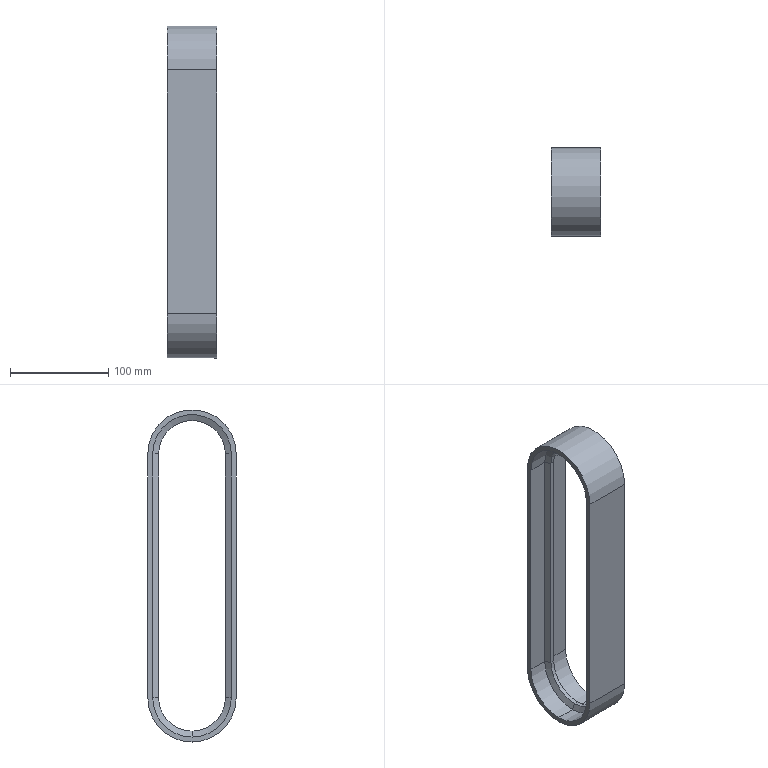Component | SolidWorks | CCD08Anti-slipBelt-1 | 1 solid | 32 faces | box 50 x 90 x 338 mm | volume 221468 mm3 | plane 14 | cylinder 12 | cone 6 | commonest cylinder face diameters 80 x6 68 x3 90 x3
STEP:
#1=COLOUR_RGB('',0.7922,0.8196,0.9333);
#2=FILL_AREA_STYLE_COLOUR('',#1);
#3=FILL_AREA_STYLE('',(#2));
#4=SURFACE_STYLE_FILL_AREA(#3);
#5=SURFACE_SIDE_STYLE('',(#4));
#6=SURFACE_STYLE_USAGE(.BOTH.,#5);
#7=PRESENTATION_STYLE_ASSIGNMENT((#6));
#8=CARTESIAN_POINT('',(-13.076,4.222,-5.236));
#9=VERTEX_POINT('',#8);
#10=CARTESIAN_POINT('',(-13.076,2.884,-3.898));
#11=VERTEX_POINT('',#10);
#12=CARTESIAN_POINT('',(-13.076,4.222,-3.898));
#13=DIRECTION('',(-1.,-0.,0.));
#14=DIRECTION('',(0.,0.,1.));
#15=AXIS2_PLACEMENT_3D('',#12,#13,#14);
#16=CIRCLE('',#15,1.339);
#17=EDGE_CURVE('',#9,#11,#16,.T.);
#18=ORIENTED_EDGE('',*,*,#17,.F.);
#19=CARTESIAN_POINT('',(-13.194,4.222,-5.472));
#20=VERTEX_POINT('',#19);
#21=CARTESIAN_POINT('',(-13.194,4.222,-5.472));
#22=DIRECTION('',(-0.4472,-0.,-0.8944));
#23=VECTOR('',#22,39.37);
#24=LINE('',#21,#23);
#25=EDGE_CURVE('',#9,#20,#24,.T.);
#26=ORIENTED_EDGE('',*,*,#25,.T.);
#27=CARTESIAN_POINT('',(-13.194,2.648,-3.898));
#28=VERTEX_POINT('',#27);
#29=CARTESIAN_POINT('',(-13.194,4.222,-3.898));
#30=DIRECTION('',(1.,0.,-0.));
#31=DIRECTION('',(0.,0.,1.));
#32=AXIS2_PLACEMENT_3D('',#29,#30,#31);
#33=CIRCLE('',#32,1.575);
#34=EDGE_CURVE('',#28,#20,#33,.T.);
#35=ORIENTED_EDGE('',*,*,#34,.F.);
#36=CARTESIAN_POINT('',(-13.194,2.648,-3.898));
#37=DIRECTION('',(0.4472,0.8944,-0.));
#38=VECTOR('',#37,39.37);
#39=LINE('',#36,#38);
#40=EDGE_CURVE('',#28,#11,#39,.T.);
#41=ORIENTED_EDGE('',*,*,#40,.T.);
#42=EDGE_LOOP('',(#18,#26,#35,#41));
#43=FACE_OUTER_BOUND('',#42,.T.);
#44=CARTESIAN_POINT('',(-13.194,4.222,-3.898));
#45=DIRECTION('',(-1.,-0.,0.));
#46=DIRECTION('',(-0.,-0.,-1.));
#47=AXIS2_PLACEMENT_3D('',#44,#45,#46);
#48=CONICAL_SURFACE('',#47,1.575,1.107);
#49=ADVANCED_FACE('',(#43),#48,.F.);
#50=CARTESIAN_POINT('',(-12.918,4.222,7.205));
#51=VERTEX_POINT('',#50);
#52=CARTESIAN_POINT('',(-12.918,2.884,5.866));
#53=VERTEX_POINT('',#52);
#54=CARTESIAN_POINT('',(-12.918,4.222,5.866));
#55=DIRECTION('',(1.,0.,-0.));
#56=DIRECTION('',(0.,0.,1.));
#57=AXIS2_PLACEMENT_3D('',#54,#55,#56);
#58=CIRCLE('',#57,1.339);
#59=EDGE_CURVE('',#51,#53,#58,.T.);
#60=ORIENTED_EDGE('',*,*,#59,.F.);
#61=CARTESIAN_POINT('',(-12.8,4.222,7.441));
#62=VERTEX_POINT('',#61);
#63=CARTESIAN_POINT('',(-12.918,4.222,7.205));
#64=DIRECTION('',(0.4472,0.,0.8944));
#65=VECTOR('',#64,39.37);
#66=LINE('',#63,#65);
#67=EDGE_CURVE('',#51,#62,#66,.T.);
#68=ORIENTED_EDGE('',*,*,#67,.T.);
#69=CARTESIAN_POINT('',(-12.8,2.648,5.866));
#70=VERTEX_POINT('',#69);
#71=CARTESIAN_POINT('',(-12.8,4.222,5.866));
#72=DIRECTION('',(1.,0.,-0.));
#73=DIRECTION('',(0.,0.,1.));
#74=AXIS2_PLACEMENT_3D('',#71,#72,#73);
#75=CIRCLE('',#74,1.575);
#76=EDGE_CURVE('',#62,#70,#75,.T.);
#77=ORIENTED_EDGE('',*,*,#76,.T.);
#78=CARTESIAN_POINT('',(-12.8,2.648,5.866));
#79=DIRECTION('',(-0.4472,0.8944,-0.));
#80=VECTOR('',#79,39.37);
#81=LINE('',#78,#80);
#82=EDGE_CURVE('',#70,#53,#81,.T.);
#83=ORIENTED_EDGE('',*,*,#82,.T.);
#84=EDGE_LOOP('',(#60,#68,#77,#83));
#85=FACE_OUTER_BOUND('',#84,.T.);
#86=CARTESIAN_POINT('',(-12.918,4.222,5.866));
#87=DIRECTION('',(1.,0.,-0.));
#88=DIRECTION('',(0.,0.,1.));
#89=AXIS2_PLACEMENT_3D('',#86,#87,#88);
#90=CONICAL_SURFACE('',#89,1.339,1.107);
#91=ADVANCED_FACE('',(#85),#90,.F.);
#92=CARTESIAN_POINT('',(-12.918,2.884,-3.898));
#93=VERTEX_POINT('',#92);
#94=CARTESIAN_POINT('',(-12.918,4.222,-5.236));
#95=VERTEX_POINT('',#94);
#96=CARTESIAN_POINT('',(-12.918,4.222,-3.898));
#97=DIRECTION('',(1.,0.,-0.));
#98=DIRECTION('',(0.,0.,1.));
#99=AXIS2_PLACEMENT_3D('',#96,#97,#98);
#100=CIRCLE('',#99,1.339);
#101=EDGE_CURVE('',#93,#95,#100,.T.);
#102=ORIENTED_EDGE('',*,*,#101,.T.);
#103=CARTESIAN_POINT('',(-12.8,4.222,-5.236));
#104=DIRECTION('',(-1.,-0.,0.));
#105=VECTOR('',#104,39.37);
#106=LINE('',#103,#105);
#107=EDGE_CURVE('',#95,#9,#106,.T.);
#108=ORIENTED_EDGE('',*,*,#107,.T.);
#109=ORIENTED_EDGE('',*,*,#17,.T.);
#110=CARTESIAN_POINT('',(-12.8,2.884,-3.898));
#111=DIRECTION('',(-1.,-0.,0.));
#112=VECTOR('',#111,39.37);
#113=LINE('',#110,#112);
#114=EDGE_CURVE('',#93,#11,#113,.T.);
#115=ORIENTED_EDGE('',*,*,#114,.F.);
#116=EDGE_LOOP('',(#102,#108,#109,#115));
#117=FACE_OUTER_BOUND('',#116,.T.);
#118=CARTESIAN_POINT('',(-12.8,4.222,-3.898));
#119=DIRECTION('',(-1.,-0.,0.));
#120=DIRECTION('',(-0.,-0.,-1.));
#121=AXIS2_PLACEMENT_3D('',#118,#119,#120);
#122=CYLINDRICAL_SURFACE('',#121,1.339);
#123=ADVANCED_FACE('',(#117),#122,.F.);
#124=CARTESIAN_POINT('',(-12.013,2.648,-3.898));
#125=VERTEX_POINT('',#124);
#126=CARTESIAN_POINT('',(-12.013,4.222,-5.472));
#127=VERTEX_POINT('',#126);
#128=CARTESIAN_POINT('',(-12.013,4.222,-3.898));
#129=DIRECTION('',(1.,0.,-0.));
#130=DIRECTION('',(0.,0.,1.));
#131=AXIS2_PLACEMENT_3D('',#128,#129,#130);
#132=CIRCLE('',#131,1.575);
#133=EDGE_CURVE('',#125,#127,#132,.T.);
#134=ORIENTED_EDGE('',*,*,#133,.T.);
#135=CARTESIAN_POINT('',(-12.8,4.222,-5.472));
#136=VERTEX_POINT('',#135);
#137=CARTESIAN_POINT('',(-12.013,4.222,-5.472));
#138=DIRECTION('',(-1.,-0.,0.));
#139=VECTOR('',#138,39.37);
#140=LINE('',#137,#139);
#141=EDGE_CURVE('',#127,#136,#140,.T.);
#142=ORIENTED_EDGE('',*,*,#141,.T.);
#143=CARTESIAN_POINT('',(-12.8,2.648,-3.898));
#144=VERTEX_POINT('',#143);
#145=CARTESIAN_POINT('',(-12.8,4.222,-3.898));
#146=DIRECTION('',(1.,0.,-0.));
#147=DIRECTION('',(0.,0.,1.));
#148=AXIS2_PLACEMENT_3D('',#145,#146,#147);
#149=CIRCLE('',#148,1.575);
#150=EDGE_CURVE('',#144,#136,#149,.T.);
#151=ORIENTED_EDGE('',*,*,#150,.F.);
#152=CARTESIAN_POINT('',(-12.013,2.648,-3.898));
#153=DIRECTION('',(-1.,-0.,0.));
#154=VECTOR('',#153,39.37);
#155=LINE('',#152,#154);
#156=EDGE_CURVE('',#125,#144,#155,.T.);
#157=ORIENTED_EDGE('',*,*,#156,.F.);
#158=EDGE_LOOP('',(#134,#142,#151,#157));
#159=FACE_OUTER_BOUND('',#158,.T.);
#160=CARTESIAN_POINT('',(-12.013,4.222,-3.898));
#161=DIRECTION('',(-1.,-0.,0.));
#162=DIRECTION('',(-0.,-0.,-1.));
#163=AXIS2_PLACEMENT_3D('',#160,#161,#162);
#164=CYLINDRICAL_SURFACE('',#163,1.575);
#165=ADVANCED_FACE('',(#159),#164,.F.);
#166=CARTESIAN_POINT('',(-12.013,4.222,-5.669));
#167=VERTEX_POINT('',#166);
#168=CARTESIAN_POINT('',(-12.013,5.994,-3.898));
#169=VERTEX_POINT('',#168);
#170=CARTESIAN_POINT('',(-12.013,4.222,-3.898));
#171=DIRECTION('',(1.,0.,-0.));
#172=DIRECTION('',(0.,0.,1.));
#173=AXIS2_PLACEMENT_3D('',#170,#171,#172);
#174=CIRCLE('',#173,1.772);
#175=EDGE_CURVE('',#167,#169,#174,.T.);
#176=ORIENTED_EDGE('',*,*,#175,.F.);
#177=CARTESIAN_POINT('',(-13.981,4.222,-5.669));
#178=VERTEX_POINT('',#177);
#179=CARTESIAN_POINT('',(-12.013,4.222,-5.669));
#180=DIRECTION('',(-1.,-0.,0.));
#181=VECTOR('',#180,39.37);
#182=LINE('',#179,#181);
#183=EDGE_CURVE('',#167,#178,#182,.T.);
#184=ORIENTED_EDGE('',*,*,#183,.T.);
#185=CARTESIAN_POINT('',(-13.981,5.994,-3.898));
#186=VERTEX_POINT('',#185);
#187=CARTESIAN_POINT('',(-13.981,4.222,-3.898));
#188=DIRECTION('',(1.,0.,-0.));
#189=DIRECTION('',(0.,0.,1.));
#190=AXIS2_PLACEMENT_3D('',#187,#188,#189);
#191=CIRCLE('',#190,1.772);
#192=EDGE_CURVE('',#178,#186,#191,.T.);
#193=ORIENTED_EDGE('',*,*,#192,.T.);
#194=CARTESIAN_POINT('',(-12.013,5.994,-3.898));
#195=DIRECTION('',(-1.,-0.,0.));
#196=VECTOR('',#195,39.37);
#197=LINE('',#194,#196);
#198=EDGE_CURVE('',#169,#186,#197,.T.);
#199=ORIENTED_EDGE('',*,*,#198,.F.);
#200=EDGE_LOOP('',(#176,#184,#193,#199));
#201=FACE_OUTER_BOUND('',#200,.T.);
#202=CARTESIAN_POINT('',(-12.013,4.222,-3.898));
#203=DIRECTION('',(-1.,-0.,0.));
#204=DIRECTION('',(-0.,-0.,-1.));
#205=AXIS2_PLACEMENT_3D('',#202,#203,#204);
#206=CYLINDRICAL_SURFACE('',#205,1.772);
#207=ADVANCED_FACE('',(#201),#206,.T.);
#208=ORIENTED_EDGE('',*,*,#34,.T.);
#209=CARTESIAN_POINT('',(-13.981,4.222,-5.472));
#210=VERTEX_POINT('',#209);
#211=CARTESIAN_POINT('',(-12.013,4.222,-5.472));
#212=DIRECTION('',(-1.,-0.,0.));
#213=VECTOR('',#212,39.37);
#214=LINE('',#211,#213);
#215=EDGE_CURVE('',#20,#210,#214,.T.);
#216=ORIENTED_EDGE('',*,*,#215,.T.);
#217=CARTESIAN_POINT('',(-13.981,2.648,-3.898));
#218=VERTEX_POINT('',#217);
#219=CARTESIAN_POINT('',(-13.981,4.222,-3.898));
#220=DIRECTION('',(1.,0.,-0.));
#221=DIRECTION('',(0.,0.,1.));
#222=AXIS2_PLACEMENT_3D('',#219,#220,#221);
#223=CIRCLE('',#222,1.575);
#224=EDGE_CURVE('',#218,#210,#223,.T.);
#225=ORIENTED_EDGE('',*,*,#224,.F.);
#226=CARTESIAN_POINT('',(-12.013,2.648,-3.898));
#227=DIRECTION('',(-1.,-0.,0.));
#228=VECTOR('',#227,39.37);
#229=LINE('',#226,#228);
#230=EDGE_CURVE('',#28,#218,#229,.T.);
#231=ORIENTED_EDGE('',*,*,#230,.F.);
#232=EDGE_LOOP('',(#208,#216,#225,#231));
#233=FACE_OUTER_BOUND('',#232,.T.);
#234=CARTESIAN_POINT('',(-12.013,4.222,-3.898));
#235=DIRECTION('',(-1.,-0.,0.));
#236=DIRECTION('',(-0.,-0.,-1.));
#237=AXIS2_PLACEMENT_3D('',#234,#235,#236);
#238=CYLINDRICAL_SURFACE('',#237,1.575);
#239=ADVANCED_FACE('',(#233),#238,.F.);
#240=ORIENTED_EDGE('',*,*,#215,.F.);
#241=CARTESIAN_POINT('',(-13.194,5.797,-3.898));
#242=VERTEX_POINT('',#241);
#243=CARTESIAN_POINT('',(-13.194,4.222,-3.898));
#244=DIRECTION('',(1.,0.,-0.));
#245=DIRECTION('',(0.,0.,1.));
#246=AXIS2_PLACEMENT_3D('',#243,#244,#245);
#247=CIRCLE('',#246,1.575);
#248=EDGE_CURVE('',#20,#242,#247,.T.);
#249=ORIENTED_EDGE('',*,*,#248,.T.);
#250=CARTESIAN_POINT('',(-13.981,5.797,-3.898));
#251=VERTEX_POINT('',#250);
#252=CARTESIAN_POINT('',(-12.013,5.797,-3.898));
#253=DIRECTION('',(-1.,-0.,0.));
#254=VECTOR('',#253,39.37);
#255=LINE('',#252,#254);
#256=EDGE_CURVE('',#242,#251,#255,.T.);
#257=ORIENTED_EDGE('',*,*,#256,.T.);
#258=CARTESIAN_POINT('',(-13.981,4.222,-3.898));
#259=DIRECTION('',(1.,0.,-0.));
#260=DIRECTION('',(0.,0.,1.));
#261=AXIS2_PLACEMENT_3D('',#258,#259,#260);
#262=CIRCLE('',#261,1.575);
#263=EDGE_CURVE('',#210,#251,#262,.T.);
#264=ORIENTED_EDGE('',*,*,#263,.F.);
#265=EDGE_LOOP('',(#240,#249,#257,#264));
#266=FACE_OUTER_BOUND('',#265,.T.);
#267=CARTESIAN_POINT('',(-12.013,4.222,-3.898));
#268=DIRECTION('',(-1.,-0.,0.));
#269=DIRECTION('',(-0.,-0.,-1.));
#270=AXIS2_PLACEMENT_3D('',#267,#268,#269);
#271=CYLINDRICAL_SURFACE('',#270,1.575);
#272=ADVANCED_FACE('',(#266),#271,.F.);
#273=ORIENTED_EDGE('',*,*,#256,.F.);
#274=CARTESIAN_POINT('',(-13.194,5.797,5.866));
#275=VERTEX_POINT('',#274);
#276=CARTESIAN_POINT('',(-13.194,5.797,-3.898));
#277=DIRECTION('',(0.,0.,1.));
#278=VECTOR('',#277,39.37);
#279=LINE('',#276,#278);
#280=EDGE_CURVE('',#242,#275,#279,.T.);
#281=ORIENTED_EDGE('',*,*,#280,.T.);
#282=CARTESIAN_POINT('',(-13.981,5.797,5.866));
#283=VERTEX_POINT('',#282);
#284=CARTESIAN_POINT('',(-12.013,5.797,5.866));
#285=DIRECTION('',(-1.,-0.,0.));
#286=VECTOR('',#285,39.37);
#287=LINE('',#284,#286);
#288=EDGE_CURVE('',#275,#283,#287,.T.);
#289=ORIENTED_EDGE('',*,*,#288,.T.);
#290=CARTESIAN_POINT('',(-13.981,5.797,-3.898));
#291=DIRECTION('',(0.,0.,1.));
#292=VECTOR('',#291,39.37);
#293=LINE('',#290,#292);
#294=EDGE_CURVE('',#251,#283,#293,.T.);
#295=ORIENTED_EDGE('',*,*,#294,.F.);
#296=EDGE_LOOP('',(#273,#281,#289,#295));
#297=FACE_OUTER_BOUND('',#296,.T.);
#298=CARTESIAN_POINT('',(-12.013,5.797,-3.898));
#299=DIRECTION('',(0.,-1.,0.));
#300=DIRECTION('',(1.,0.,-0.));
#301=AXIS2_PLACEMENT_3D('',#298,#299,#300);
#302=PLANE('',#301);
#303=ADVANCED_FACE('',(#297),#302,.T.);
#304=ORIENTED_EDGE('',*,*,#288,.F.);
#305=CARTESIAN_POINT('',(-13.194,2.648,5.866));
#306=VERTEX_POINT('',#305);
#307=CARTESIAN_POINT('',(-13.194,4.222,5.866));
#308=DIRECTION('',(1.,0.,-0.));
#309=DIRECTION('',(0.,0.,1.));
#310=AXIS2_PLACEMENT_3D('',#307,#308,#309);
#311=CIRCLE('',#310,1.575);
#312=EDGE_CURVE('',#275,#306,#311,.T.);
#313=ORIENTED_EDGE('',*,*,#312,.T.);
#314=CARTESIAN_POINT('',(-13.981,2.648,5.866));
#315=VERTEX_POINT('',#314);
#316=CARTESIAN_POINT('',(-12.013,2.648,5.866));
#317=DIRECTION('',(-1.,-0.,0.));
#318=VECTOR('',#317,39.37);
#319=LINE('',#316,#318);
#320=EDGE_CURVE('',#306,#315,#319,.T.);
#321=ORIENTED_EDGE('',*,*,#320,.T.);
#322=CARTESIAN_POINT('',(-13.981,4.222,5.866));
#323=DIRECTION('',(1.,0.,-0.));
#324=DIRECTION('',(0.,0.,1.));
#325=AXIS2_PLACEMENT_3D('',#322,#323,#324);
#326=CIRCLE('',#325,1.575);
#327=EDGE_CURVE('',#283,#315,#326,.T.);
#328=ORIENTED_EDGE('',*,*,#327,.F.);
#329=EDGE_LOOP('',(#304,#313,#321,#328));
#330=FACE_OUTER_BOUND('',#329,.T.);
#331=CARTESIAN_POINT('',(-12.013,4.222,5.866));
#332=DIRECTION('',(-1.,-0.,0.));
#333=DIRECTION('',(-0.,-0.,-1.));
#334=AXIS2_PLACEMENT_3D('',#331,#332,#333);
#335=CYLINDRICAL_SURFACE('',#334,1.575);
#336=ADVANCED_FACE('',(#330),#335,.F.);
#337=ORIENTED_EDGE('',*,*,#320,.F.);
#338=CARTESIAN_POINT('',(-13.194,2.648,-3.898));
#339=DIRECTION('',(-0.,-0.,-1.));
#340=VECTOR('',#339,39.37);
#341=LINE('',#338,#340);
#342=EDGE_CURVE('',#306,#28,#341,.T.);
#343=ORIENTED_EDGE('',*,*,#342,.T.);
#344=ORIENTED_EDGE('',*,*,#230,.T.);
#345=CARTESIAN_POINT('',(-13.981,2.648,-3.898));
#346=DIRECTION('',(-0.,-0.,-1.));
#347=VECTOR('',#346,39.37);
#348=LINE('',#345,#347);
#349=EDGE_CURVE('',#315,#218,#348,.T.);
#350=ORIENTED_EDGE('',*,*,#349,.F.);
#351=EDGE_LOOP('',(#337,#343,#344,#350));
#352=FACE_OUTER_BOUND('',#351,.T.);
#353=CARTESIAN_POINT('',(-12.013,2.648,-3.898));
#354=DIRECTION('',(-0.,1.,-0.));
#355=DIRECTION('',(-1.,-0.,0.));
#356=AXIS2_PLACEMENT_3D('',#353,#354,#355);
#357=PLANE('',#356);
#358=ADVANCED_FACE('',(#352),#357,.T.);
#359=CARTESIAN_POINT('',(-12.013,2.451,-3.898));
#360=VERTEX_POINT('',#359);
#361=CARTESIAN_POINT('',(-12.013,4.222,-3.898));
#362=DIRECTION('',(1.,0.,-0.));
#363=DIRECTION('',(0.,0.,1.));
#364=AXIS2_PLACEMENT_3D('',#361,#362,#363);
#365=CIRCLE('',#364,1.772);
#366=EDGE_CURVE('',#360,#167,#365,.T.);
#367=ORIENTED_EDGE('',*,*,#366,.T.);
#368=ORIENTED_EDGE('',*,*,#175,.T.);
#369=CARTESIAN_POINT('',(-12.013,5.994,5.866));
#370=VERTEX_POINT('',#369);
#371=CARTESIAN_POINT('',(-12.013,5.994,-3.898));
#372=DIRECTION('',(0.,0.,1.));
#373=VECTOR('',#372,39.37);
#374=LINE('',#371,#373);
#375=EDGE_CURVE('',#169,#370,#374,.T.);
#376=ORIENTED_EDGE('',*,*,#375,.T.);
#377=CARTESIAN_POINT('',(-12.013,2.451,5.866));
#378=VERTEX_POINT('',#377);
#379=CARTESIAN_POINT('',(-12.013,4.222,5.866));
#380=DIRECTION('',(1.,0.,-0.));
#381=DIRECTION('',(0.,0.,1.));
#382=AXIS2_PLACEMENT_3D('',#379,#380,#381);
#383=CIRCLE('',#382,1.772);
#384=EDGE_CURVE('',#370,#378,#383,.T.);
#385=ORIENTED_EDGE('',*,*,#384,.T.);
#386=CARTESIAN_POINT('',(-12.013,2.451,-3.898));
#387=DIRECTION('',(-0.,-0.,-1.));
#388=VECTOR('',#387,39.37);
#389=LINE('',#386,#388);
#390=EDGE_CURVE('',#378,#360,#389,.T.);
#391=ORIENTED_EDGE('',*,*,#390,.T.);
#392=EDGE_LOOP('',(#367,#368,#376,#385,#391));
#393=FACE_OUTER_BOUND('',#392,.T.);
#394=CARTESIAN_POINT('',(-12.013,5.797,-3.898));
#395=VERTEX_POINT('',#394);
#396=CARTESIAN_POINT('',(-12.013,5.797,5.866));
#397=VERTEX_POINT('',#396);
#398=CARTESIAN_POINT('',(-12.013,5.797,-3.898));
#399=DIRECTION('',(0.,0.,1.));
#400=VECTOR('',#399,39.37);
#401=LINE('',#398,#400);
#402=EDGE_CURVE('',#395,#397,#401,.T.);
#403=ORIENTED_EDGE('',*,*,#402,.F.);
#404=CARTESIAN_POINT('',(-12.013,4.222,-3.898));
#405=DIRECTION('',(1.,0.,-0.));
#406=DIRECTION('',(0.,0.,1.));
#407=AXIS2_PLACEMENT_3D('',#404,#405,#406);
#408=CIRCLE('',#407,1.575);
#409=EDGE_CURVE('',#127,#395,#408,.T.);
#410=ORIENTED_EDGE('',*,*,#409,.F.);
#411=ORIENTED_EDGE('',*,*,#133,.F.);
#412=CARTESIAN_POINT('',(-12.013,2.648,5.866));
#413=VERTEX_POINT('',#412);
#414=CARTESIAN_POINT('',(-12.013,2.648,-3.898));
#415=DIRECTION('',(-0.,-0.,-1.));
#416=VECTOR('',#415,39.37);
#417=LINE('',#414,#416);
#418=EDGE_CURVE('',#413,#125,#417,.T.);
#419=ORIENTED_EDGE('',*,*,#418,.F.);
#420=CARTESIAN_POINT('',(-12.013,4.222,5.866));
#421=DIRECTION('',(1.,0.,-0.));
#422=DIRECTION('',(0.,0.,1.));
#423=AXIS2_PLACEMENT_3D('',#420,#421,#422);
#424=CIRCLE('',#423,1.575);
#425=EDGE_CURVE('',#397,#413,#424,.T.);
#426=ORIENTED_EDGE('',*,*,#425,.F.);
#427=EDGE_LOOP('',(#403,#410,#411,#419,#426));
#428=FACE_BOUND('',#427,.T.);
#429=CARTESIAN_POINT('',(-12.013,4.222,-3.898));
#430=DIRECTION('',(1.,0.,-0.));
#431=DIRECTION('',(0.,0.,1.));
#432=AXIS2_PLACEMENT_3D('',#429,#430,#431);
#433=PLANE('',#432);
#434=ADVANCED_FACE('',(#393,#428),#433,.T.);
#435=CARTESIAN_POINT('',(-13.981,2.451,-3.898));
#436=VERTEX_POINT('',#435);
#437=CARTESIAN_POINT('',(-13.981,4.222,-3.898));
#438=DIRECTION('',(1.,0.,-0.));
#439=DIRECTION('',(0.,0.,1.));
#440=AXIS2_PLACEMENT_3D('',#437,#438,#439);
#441=CIRCLE('',#440,1.772);
#442=EDGE_CURVE('',#436,#178,#441,.T.);
#443=ORIENTED_EDGE('',*,*,#442,.F.);
#444=CARTESIAN_POINT('',(-13.981,2.451,5.866));
#445=VERTEX_POINT('',#444);
#446=CARTESIAN_POINT('',(-13.981,2.451,-3.898));
#447=DIRECTION('',(-0.,-0.,-1.));
#448=VECTOR('',#447,39.37);
#449=LINE('',#446,#448);
#450=EDGE_CURVE('',#445,#436,#449,.T.);
#451=ORIENTED_EDGE('',*,*,#450,.F.);
#452=CARTESIAN_POINT('',(-13.981,5.994,5.866));
#453=VERTEX_POINT('',#452);
#454=CARTESIAN_POINT('',(-13.981,4.222,5.866));
#455=DIRECTION('',(1.,0.,-0.));
#456=DIRECTION('',(0.,0.,1.));
#457=AXIS2_PLACEMENT_3D('',#454,#455,#456);
#458=CIRCLE('',#457,1.772);
#459=EDGE_CURVE('',#453,#445,#458,.T.);
#460=ORIENTED_EDGE('',*,*,#459,.F.);
#461=CARTESIAN_POINT('',(-13.981,5.994,-3.898));
#462=DIRECTION('',(0.,0.,1.));
#463=VECTOR('',#462,39.37);
#464=LINE('',#461,#463);
#465=EDGE_CURVE('',#186,#453,#464,.T.);
#466=ORIENTED_EDGE('',*,*,#465,.F.);
#467=ORIENTED_EDGE('',*,*,#192,.F.);
#468=EDGE_LOOP('',(#443,#451,#460,#466,#467));
#469=FACE_OUTER_BOUND('',#468,.T.);
#470=ORIENTED_EDGE('',*,*,#224,.T.);
#471=ORIENTED_EDGE('',*,*,#263,.T.);
#472=ORIENTED_EDGE('',*,*,#294,.T.);
#473=ORIENTED_EDGE('',*,*,#327,.T.);
#474=ORIENTED_EDGE('',*,*,#349,.T.);
#475=EDGE_LOOP('',(#470,#471,#472,#473,#474));
#476=FACE_BOUND('',#475,.T.);
#477=CARTESIAN_POINT('',(-13.981,4.222,-3.898));
#478=DIRECTION('',(1.,0.,-0.));
#479=DIRECTION('',(0.,0.,1.));
#480=AXIS2_PLACEMENT_3D('',#477,#478,#479);
#481=PLANE('',#480);
#482=ADVANCED_FACE('',(#469,#476),#481,.F.);
#483=ORIENTED_EDGE('',*,*,#183,.F.);
#484=ORIENTED_EDGE('',*,*,#366,.F.);
#485=CARTESIAN_POINT('',(-12.013,2.451,-3.898));
#486=DIRECTION('',(-1.,-0.,0.));
#487=VECTOR('',#486,39.37);
#488=LINE('',#485,#487);
#489=EDGE_CURVE('',#360,#436,#488,.T.);
#490=ORIENTED_EDGE('',*,*,#489,.T.);
#491=ORIENTED_EDGE('',*,*,#442,.T.);
#492=EDGE_LOOP('',(#483,#484,#490,#491));
#493=FACE_OUTER_BOUND('',#492,.T.);
#494=CARTESIAN_POINT('',(-12.013,4.222,-3.898));
#495=DIRECTION('',(-1.,-0.,0.));
#496=DIRECTION('',(-0.,-0.,-1.));
#497=AXIS2_PLACEMENT_3D('',#494,#495,#496);
#498=CYLINDRICAL_SURFACE('',#497,1.772);
#499=ADVANCED_FACE('',(#493),#498,.T.);
#500=ORIENTED_EDGE('',*,*,#465,.T.);
#501=CARTESIAN_POINT('',(-12.013,5.994,5.866));
#502=DIRECTION('',(-1.,-0.,0.));
#503=VECTOR('',#502,39.37);
#504=LINE('',#501,#503);
#505=EDGE_CURVE('',#370,#453,#504,.T.);
#506=ORIENTED_EDGE('',*,*,#505,.F.);
#507=ORIENTED_EDGE('',*,*,#375,.F.);
#508=ORIENTED_EDGE('',*,*,#198,.T.);
#509=EDGE_LOOP('',(#500,#506,#507,#508));
#510=FACE_OUTER_BOUND('',#509,.T.);
#511=CARTESIAN_POINT('',(-12.013,5.994,-3.898));
#512=DIRECTION('',(0.,-1.,0.));
#513=DIRECTION('',(1.,0.,-0.));
#514=AXIS2_PLACEMENT_3D('',#511,#512,#513);
#515=PLANE('',#514);
#516=ADVANCED_FACE('',(#510),#515,.F.);
#517=ORIENTED_EDGE('',*,*,#459,.T.);
#518=CARTESIAN_POINT('',(-12.013,2.451,5.866));
#519=DIRECTION('',(-1.,-0.,0.));
#520=VECTOR('',#519,39.37);
#521=LINE('',#518,#520);
#522=EDGE_CURVE('',#378,#445,#521,.T.);
#523=ORIENTED_EDGE('',*,*,#522,.F.);
#524=ORIENTED_EDGE('',*,*,#384,.F.);
#525=ORIENTED_EDGE('',*,*,#505,.T.);
#526=EDGE_LOOP('',(#517,#523,#524,#525));
#527=FACE_OUTER_BOUND('',#526,.T.);
#528=CARTESIAN_POINT('',(-12.013,4.222,5.866));
#529=DIRECTION('',(-1.,-0.,0.));
#530=DIRECTION('',(-0.,-0.,-1.));
#531=AXIS2_PLACEMENT_3D('',#528,#529,#530);
#532=CYLINDRICAL_SURFACE('',#531,1.772);
#533=ADVANCED_FACE('',(#527),#532,.T.);
#534=ORIENTED_EDGE('',*,*,#450,.T.);
#535=ORIENTED_EDGE('',*,*,#489,.F.);
#536=ORIENTED_EDGE('',*,*,#390,.F.);
#537=ORIENTED_EDGE('',*,*,#522,.T.);
#538=EDGE_LOOP('',(#534,#535,#536,#537));
#539=FACE_OUTER_BOUND('',#538,.T.);
#540=CARTESIAN_POINT('',(-12.013,2.451,-3.898));
#541=DIRECTION('',(-0.,1.,-0.));
#542=DIRECTION('',(-1.,-0.,0.));
#543=AXIS2_PLACEMENT_3D('',#540,#541,#542);
#544=PLANE('',#543);
#545=ADVANCED_FACE('',(#539),#544,.F.);
#546=ORIENTED_EDGE('',*,*,#141,.F.);
#547=ORIENTED_EDGE('',*,*,#409,.T.);
#548=CARTESIAN_POINT('',(-12.8,5.797,-3.898));
#549=VERTEX_POINT('',#548);
#550=CARTESIAN_POINT('',(-12.013,5.797,-3.898));
#551=DIRECTION('',(-1.,-0.,0.));
#552=VECTOR('',#551,39.37);
#553=LINE('',#550,#552);
#554=EDGE_CURVE('',#395,#549,#553,.T.);
#555=ORIENTED_EDGE('',*,*,#554,.T.);
#556=CARTESIAN_POINT('',(-12.8,4.222,-3.898));
#557=DIRECTION('',(1.,0.,-0.));
#558=DIRECTION('',(0.,0.,1.));
#559=AXIS2_PLACEMENT_3D('',#556,#557,#558);
#560=CIRCLE('',#559,1.575);
#561=EDGE_CURVE('',#136,#549,#560,.T.);
#562=ORIENTED_EDGE('',*,*,#561,.F.);
#563=EDGE_LOOP('',(#546,#547,#555,#562));
#564=FACE_OUTER_BOUND('',#563,.T.);
#565=CARTESIAN_POINT('',(-12.013,4.222,-3.898));
#566=DIRECTION('',(-1.,-0.,0.));
#567=DIRECTION('',(-0.,-0.,-1.));
#568=AXIS2_PLACEMENT_3D('',#565,#566,#567);
#569=CYLINDRICAL_SURFACE('',#568,1.575);
#570=ADVANCED_FACE('',(#564),#569,.F.);
#571=CARTESIAN_POINT('',(-12.8,5.797,5.866));
#572=VERTEX_POINT('',#571);
#573=CARTESIAN_POINT('',(-12.8,5.797,-3.898));
#574=DIRECTION('',(0.,0.,1.));
#575=VECTOR('',#574,39.37);
#576=LINE('',#573,#575);
#577=EDGE_CURVE('',#549,#572,#576,.T.);
#578=ORIENTED_EDGE('',*,*,#577,.F.);
#579=ORIENTED_EDGE('',*,*,#554,.F.);
#580=ORIENTED_EDGE('',*,*,#402,.T.);
#581=CARTESIAN_POINT('',(-12.013,5.797,5.866));
#582=DIRECTION('',(-1.,-0.,0.));
#583=VECTOR('',#582,39.37);
#584=LINE('',#581,#583);
#585=EDGE_CURVE('',#397,#572,#584,.T.);
#586=ORIENTED_EDGE('',*,*,#585,.T.);
#587=EDGE_LOOP('',(#578,#579,#580,#586));
#588=FACE_OUTER_BOUND('',#587,.T.);
#589=CARTESIAN_POINT('',(-12.013,5.797,-3.898));
#590=DIRECTION('',(0.,-1.,0.));
#591=DIRECTION('',(1.,0.,-0.));
#592=AXIS2_PLACEMENT_3D('',#589,#590,#591);
#593=PLANE('',#592);
#594=ADVANCED_FACE('',(#588),#593,.T.);
#595=CARTESIAN_POINT('',(-12.8,4.222,5.866));
#596=DIRECTION('',(1.,0.,-0.));
#597=DIRECTION('',(0.,0.,1.));
#598=AXIS2_PLACEMENT_3D('',#595,#596,#597);
#599=CIRCLE('',#598,1.575);
#600=EDGE_CURVE('',#572,#62,#599,.T.);
#601=ORIENTED_EDGE('',*,*,#600,.F.);
#602=ORIENTED_EDGE('',*,*,#585,.F.);
#603=ORIENTED_EDGE('',*,*,#425,.T.);
#604=CARTESIAN_POINT('',(-12.013,2.648,5.866));
#605=DIRECTION('',(-1.,-0.,0.));
#606=VECTOR('',#605,39.37);
#607=LINE('',#604,#606);
#608=EDGE_CURVE('',#413,#70,#607,.T.);
#609=ORIENTED_EDGE('',*,*,#608,.T.);
#610=ORIENTED_EDGE('',*,*,#76,.F.);
#611=EDGE_LOOP('',(#601,#602,#603,#609,#610));
#612=FACE_OUTER_BOUND('',#611,.T.);
#613=CARTESIAN_POINT('',(-12.013,4.222,5.866));
#614=DIRECTION('',(-1.,-0.,0.));
#615=DIRECTION('',(-0.,-0.,-1.));
#616=AXIS2_PLACEMENT_3D('',#613,#614,#615);
#617=CYLINDRICAL_SURFACE('',#616,1.575);
#618=ADVANCED_FACE('',(#612),#617,.F.);
#619=CARTESIAN_POINT('',(-12.8,2.648,-3.898));
#620=DIRECTION('',(-0.,-0.,-1.));
#621=VECTOR('',#620,39.37);
#622=LINE('',#619,#621);
#623=EDGE_CURVE('',#70,#144,#622,.T.);
#624=ORIENTED_EDGE('',*,*,#623,.F.);
#625=ORIENTED_EDGE('',*,*,#608,.F.);
#626=ORIENTED_EDGE('',*,*,#418,.T.);
#627=ORIENTED_EDGE('',*,*,#156,.T.);
#628=EDGE_LOOP('',(#624,#625,#626,#627));
#629=FACE_OUTER_BOUND('',#628,.T.);
#630=CARTESIAN_POINT('',(-12.013,2.648,-3.898));
#631=DIRECTION('',(-0.,1.,-0.));
#632=DIRECTION('',(-1.,-0.,0.));
#633=AXIS2_PLACEMENT_3D('',#630,#631,#632);
#634=PLANE('',#633);
#635=ADVANCED_FACE('',(#629),#634,.T.);
#636=ORIENTED_EDGE('',*,*,#107,.F.);
#637=CARTESIAN_POINT('',(-12.918,5.561,-3.898));
#638=VERTEX_POINT('',#637);
#639=CARTESIAN_POINT('',(-12.918,4.222,-3.898));
#640=DIRECTION('',(1.,0.,-0.));
#641=DIRECTION('',(0.,0.,1.));
#642=AXIS2_PLACEMENT_3D('',#639,#640,#641);
#643=CIRCLE('',#642,1.339);
#644=EDGE_CURVE('',#95,#638,#643,.T.);
#645=ORIENTED_EDGE('',*,*,#644,.T.);
#646=CARTESIAN_POINT('',(-13.076,5.561,-3.898));
#647=VERTEX_POINT('',#646);
#648=CARTESIAN_POINT('',(-12.8,5.561,-3.898));
#649=DIRECTION('',(-1.,-0.,0.));
#650=VECTOR('',#649,39.37);
#651=LINE('',#648,#650);
#652=EDGE_CURVE('',#638,#647,#651,.T.);
#653=ORIENTED_EDGE('',*,*,#652,.T.);
#654=CARTESIAN_POINT('',(-13.076,4.222,-3.898));
#655=DIRECTION('',(-1.,-0.,0.));
#656=DIRECTION('',(0.,0.,1.));
#657=AXIS2_PLACEMENT_3D('',#654,#655,#656);
#658=CIRCLE('',#657,1.339);
#659=EDGE_CURVE('',#647,#9,#658,.T.);
#660=ORIENTED_EDGE('',*,*,#659,.T.);
#661=EDGE_LOOP('',(#636,#645,#653,#660));
#662=FACE_OUTER_BOUND('',#661,.T.);
#663=CARTESIAN_POINT('',(-12.8,4.222,-3.898));
#664=DIRECTION('',(-1.,-0.,0.));
#665=DIRECTION('',(-0.,-0.,-1.));
#666=AXIS2_PLACEMENT_3D('',#663,#664,#665);
#667=CYLINDRICAL_SURFACE('',#666,1.339);
#668=ADVANCED_FACE('',(#662),#667,.F.);
#669=CARTESIAN_POINT('',(-12.918,5.561,5.866));
#670=VERTEX_POINT('',#669);
#671=CARTESIAN_POINT('',(-13.076,5.561,5.866));
#672=VERTEX_POINT('',#671);
#673=CARTESIAN_POINT('',(-12.8,5.561,5.866));
#674=DIRECTION('',(-1.,-0.,0.));
#675=VECTOR('',#674,39.37);
#676=LINE('',#673,#675);
#677=EDGE_CURVE('',#670,#672,#676,.T.);
#678=ORIENTED_EDGE('',*,*,#677,.T.);
#679=CARTESIAN_POINT('',(-13.076,5.561,-3.898));
#680=DIRECTION('',(-0.,-0.,-1.));
#681=VECTOR('',#680,39.37);
#682=LINE('',#679,#681);
#683=EDGE_CURVE('',#672,#647,#682,.T.);
#684=ORIENTED_EDGE('',*,*,#683,.T.);
#685=ORIENTED_EDGE('',*,*,#652,.F.);
#686=CARTESIAN_POINT('',(-12.918,5.561,-3.898));
#687=DIRECTION('',(0.,0.,1.));
#688=VECTOR('',#687,39.37);
#689=LINE('',#686,#688);
#690=EDGE_CURVE('',#638,#670,#689,.T.);
#691=ORIENTED_EDGE('',*,*,#690,.T.);
#692=EDGE_LOOP('',(#678,#684,#685,#691));
#693=FACE_OUTER_BOUND('',#692,.T.);
#694=CARTESIAN_POINT('',(-12.8,5.561,-3.898));
#695=DIRECTION('',(0.,-1.,0.));
#696=DIRECTION('',(1.,0.,-0.));
#697=AXIS2_PLACEMENT_3D('',#694,#695,#696);
#698=PLANE('',#697);
#699=ADVANCED_FACE('',(#693),#698,.T.);
#700=CARTESIAN_POINT('',(-13.076,2.884,5.866));
#701=VERTEX_POINT('',#700);
#702=CARTESIAN_POINT('',(-12.8,2.884,5.866));
#703=DIRECTION('',(-1.,-0.,0.));
#704=VECTOR('',#703,39.37);
#705=LINE('',#702,#704);
#706=EDGE_CURVE('',#53,#701,#705,.T.);
#707=ORIENTED_EDGE('',*,*,#706,.T.);
#708=CARTESIAN_POINT('',(-13.076,4.222,5.866));
#709=DIRECTION('',(-1.,-0.,0.));
#710=DIRECTION('',(0.,0.,1.));
#711=AXIS2_PLACEMENT_3D('',#708,#709,#710);
#712=CIRCLE('',#711,1.339);
#713=EDGE_CURVE('',#701,#672,#712,.T.);
#714=ORIENTED_EDGE('',*,*,#713,.T.);
#715=ORIENTED_EDGE('',*,*,#677,.F.);
#716=CARTESIAN_POINT('',(-12.918,4.222,5.866));
#717=DIRECTION('',(1.,0.,-0.));
#718=DIRECTION('',(0.,0.,1.));
#719=AXIS2_PLACEMENT_3D('',#716,#717,#718);
#720=CIRCLE('',#719,1.339);
#721=EDGE_CURVE('',#670,#51,#720,.T.);
#722=ORIENTED_EDGE('',*,*,#721,.T.);
#723=ORIENTED_EDGE('',*,*,#59,.T.);
#724=EDGE_LOOP('',(#707,#714,#715,#722,#723));
#725=FACE_OUTER_BOUND('',#724,.T.);
#726=CARTESIAN_POINT('',(-12.8,4.222,5.866));
#727=DIRECTION('',(-1.,-0.,0.));
#728=DIRECTION('',(-0.,-0.,-1.));
#729=AXIS2_PLACEMENT_3D('',#726,#727,#728);
#730=CYLINDRICAL_SURFACE('',#729,1.339);
#731=ADVANCED_FACE('',(#725),#730,.F.);
#732=ORIENTED_EDGE('',*,*,#114,.T.);
#733=CARTESIAN_POINT('',(-13.076,2.884,5.866));
#734=DIRECTION('',(0.,0.,1.));
#735=VECTOR('',#734,39.37);
#736=LINE('',#733,#735);
#737=EDGE_CURVE('',#11,#701,#736,.T.);
#738=ORIENTED_EDGE('',*,*,#737,.T.);
#739=ORIENTED_EDGE('',*,*,#706,.F.);
#740=CARTESIAN_POINT('',(-12.918,2.884,-3.898));
#741=DIRECTION('',(-0.,-0.,-1.));
#742=VECTOR('',#741,39.37);
#743=LINE('',#740,#742);
#744=EDGE_CURVE('',#53,#93,#743,.T.);
#745=ORIENTED_EDGE('',*,*,#744,.T.);
#746=EDGE_LOOP('',(#732,#738,#739,#745));
#747=FACE_OUTER_BOUND('',#746,.T.);
#748=CARTESIAN_POINT('',(-12.8,2.884,-3.898));
#749=DIRECTION('',(-0.,1.,-0.));
#750=DIRECTION('',(-1.,-0.,0.));
#751=AXIS2_PLACEMENT_3D('',#748,#749,#750);
#752=PLANE('',#751);
#753=ADVANCED_FACE('',(#747),#752,.T.);
#754=CARTESIAN_POINT('',(-12.8,2.648,-3.898));
#755=DIRECTION('',(-0.4472,0.8944,-0.));
#756=VECTOR('',#755,39.37);
#757=LINE('',#754,#756);
#758=EDGE_CURVE('',#144,#93,#757,.T.);
#759=ORIENTED_EDGE('',*,*,#758,.F.);
#760=ORIENTED_EDGE('',*,*,#150,.T.);
#761=ORIENTED_EDGE('',*,*,#561,.T.);
#762=CARTESIAN_POINT('',(-12.918,5.561,-3.898));
#763=DIRECTION('',(0.4472,0.8944,-0.));
#764=VECTOR('',#763,39.37);
#765=LINE('',#762,#764);
#766=EDGE_CURVE('',#638,#549,#765,.T.);
#767=ORIENTED_EDGE('',*,*,#766,.F.);
#768=ORIENTED_EDGE('',*,*,#644,.F.);
#769=ORIENTED_EDGE('',*,*,#101,.F.);
#770=EDGE_LOOP('',(#759,#760,#761,#767,#768,#769));
#771=FACE_OUTER_BOUND('',#770,.T.);
#772=CARTESIAN_POINT('',(-12.918,4.222,-3.898));
#773=DIRECTION('',(1.,0.,-0.));
#774=DIRECTION('',(0.,0.,1.));
#775=AXIS2_PLACEMENT_3D('',#772,#773,#774);
#776=CONICAL_SURFACE('',#775,1.339,1.107);
#777=ADVANCED_FACE('',(#771),#776,.F.);
#778=ORIENTED_EDGE('',*,*,#766,.T.);
#779=ORIENTED_EDGE('',*,*,#577,.T.);
#780=CARTESIAN_POINT('',(-12.918,5.561,5.866));
#781=DIRECTION('',(0.4472,0.8944,-0.));
#782=VECTOR('',#781,39.37);
#783=LINE('',#780,#782);
#784=EDGE_CURVE('',#670,#572,#783,.T.);
#785=ORIENTED_EDGE('',*,*,#784,.F.);
#786=ORIENTED_EDGE('',*,*,#690,.F.);
#787=EDGE_LOOP('',(#778,#779,#785,#786));
#788=FACE_OUTER_BOUND('',#787,.T.);
#789=CARTESIAN_POINT('',(-12.918,5.561,-3.898));
#790=DIRECTION('',(-0.8944,0.4472,-0.));
#791=DIRECTION('',(0.,0.,1.));
#792=AXIS2_PLACEMENT_3D('',#789,#790,#791);
#793=PLANE('',#792);
#794=ADVANCED_FACE('',(#788),#793,.F.);
#795=ORIENTED_EDGE('',*,*,#758,.T.);
#796=ORIENTED_EDGE('',*,*,#744,.F.);
#797=ORIENTED_EDGE('',*,*,#82,.F.);
#798=ORIENTED_EDGE('',*,*,#623,.T.);
#799=EDGE_LOOP('',(#795,#796,#797,#798));
#800=FACE_OUTER_BOUND('',#799,.T.);
#801=CARTESIAN_POINT('',(-12.918,2.884,-3.898));
#802=DIRECTION('',(-0.8944,-0.4472,0.));
#803=DIRECTION('',(-0.,-0.,-1.));
#804=AXIS2_PLACEMENT_3D('',#801,#802,#803);
#805=PLANE('',#804);
#806=ADVANCED_FACE('',(#800),#805,.F.);
#807=ORIENTED_EDGE('',*,*,#67,.F.);
#808=ORIENTED_EDGE('',*,*,#721,.F.);
#809=ORIENTED_EDGE('',*,*,#784,.T.);
#810=ORIENTED_EDGE('',*,*,#600,.T.);
#811=EDGE_LOOP('',(#807,#808,#809,#810));
#812=FACE_OUTER_BOUND('',#811,.T.);
#813=CARTESIAN_POINT('',(-12.918,4.222,5.866));
#814=DIRECTION('',(1.,0.,-0.));
#815=DIRECTION('',(0.,0.,1.));
#816=AXIS2_PLACEMENT_3D('',#813,#814,#815);
#817=CONICAL_SURFACE('',#816,1.339,1.107);
#818=ADVANCED_FACE('',(#812),#817,.F.);
#819=CARTESIAN_POINT('',(-13.076,2.884,5.866));
#820=DIRECTION('',(-0.4472,-0.8944,0.));
#821=VECTOR('',#820,39.37);
#822=LINE('',#819,#821);
#823=EDGE_CURVE('',#701,#306,#822,.T.);
#824=ORIENTED_EDGE('',*,*,#823,.F.);
#825=ORIENTED_EDGE('',*,*,#737,.F.);
#826=ORIENTED_EDGE('',*,*,#40,.F.);
#827=ORIENTED_EDGE('',*,*,#342,.F.);
#828=EDGE_LOOP('',(#824,#825,#826,#827));
#829=FACE_OUTER_BOUND('',#828,.T.);
#830=CARTESIAN_POINT('',(-13.194,2.648,-3.898));
#831=DIRECTION('',(-0.8944,0.4472,-0.));
#832=DIRECTION('',(0.,0.,1.));
#833=AXIS2_PLACEMENT_3D('',#830,#831,#832);
#834=PLANE('',#833);
#835=ADVANCED_FACE('',(#829),#834,.T.);
#836=ORIENTED_EDGE('',*,*,#25,.F.);
#837=ORIENTED_EDGE('',*,*,#659,.F.);
#838=CARTESIAN_POINT('',(-13.194,5.797,-3.898));
#839=DIRECTION('',(0.4472,-0.8944,0.));
#840=VECTOR('',#839,39.37);
#841=LINE('',#838,#840);
#842=EDGE_CURVE('',#242,#647,#841,.T.);
#843=ORIENTED_EDGE('',*,*,#842,.F.);
#844=ORIENTED_EDGE('',*,*,#248,.F.);
#845=EDGE_LOOP('',(#836,#837,#843,#844));
#846=FACE_OUTER_BOUND('',#845,.T.);
#847=CARTESIAN_POINT('',(-13.194,4.222,-3.898));
#848=DIRECTION('',(-1.,-0.,0.));
#849=DIRECTION('',(-0.,-0.,-1.));
#850=AXIS2_PLACEMENT_3D('',#847,#848,#849);
#851=CONICAL_SURFACE('',#850,1.575,1.107);
#852=ADVANCED_FACE('',(#846),#851,.F.);
#853=ORIENTED_EDGE('',*,*,#823,.T.);
#854=ORIENTED_EDGE('',*,*,#312,.F.);
#855=CARTESIAN_POINT('',(-13.076,5.561,5.866));
#856=DIRECTION('',(-0.4472,0.8944,-0.));
#857=VECTOR('',#856,39.37);
#858=LINE('',#855,#857);
#859=EDGE_CURVE('',#672,#275,#858,.T.);
#860=ORIENTED_EDGE('',*,*,#859,.F.);
#861=ORIENTED_EDGE('',*,*,#713,.F.);
#862=EDGE_LOOP('',(#853,#854,#860,#861));
#863=FACE_OUTER_BOUND('',#862,.T.);
#864=CARTESIAN_POINT('',(-13.194,4.222,5.866));
#865=DIRECTION('',(-1.,-0.,0.));
#866=DIRECTION('',(-0.,-0.,-1.));
#867=AXIS2_PLACEMENT_3D('',#864,#865,#866);
#868=CONICAL_SURFACE('',#867,1.575,1.107);
#869=ADVANCED_FACE('',(#863),#868,.F.);
#870=ORIENTED_EDGE('',*,*,#842,.T.);
#871=ORIENTED_EDGE('',*,*,#683,.F.);
#872=ORIENTED_EDGE('',*,*,#859,.T.);
#873=ORIENTED_EDGE('',*,*,#280,.F.);
#874=EDGE_LOOP('',(#870,#871,#872,#873));
#875=FACE_OUTER_BOUND('',#874,.T.);
#876=CARTESIAN_POINT('',(-13.194,5.797,-3.898));
#877=DIRECTION('',(-0.8944,-0.4472,0.));
#878=DIRECTION('',(-0.,-0.,-1.));
#879=AXIS2_PLACEMENT_3D('',#876,#877,#878);
#880=PLANE('',#879);
#881=ADVANCED_FACE('',(#875),#880,.T.);
#882=CLOSED_SHELL('',(#49,#91,#123,#165,#207,#239,#272,#303,#336,#358,#434,#482,#499,#516,#533,#545,#570,#594,#618,#635,#668,#699,#731,#753,#777,#794,#806,#818,#835,#852,#869,#881));
#883=MANIFOLD_SOLID_BREP('',#882);
#884=STYLED_ITEM('',(#7),#883);
#885=PRESENTATION_LAYER_ASSIGNMENT('','',(#884));
#886=CARTESIAN_POINT('',(0.,0.,0.));
#887=DIRECTION('',(0.,0.,1.));
#888=DIRECTION('',(1.,0.,0.));
#889=AXIS2_PLACEMENT_3D('',#886,#887,#888);
#890=(LENGTH_UNIT()NAMED_UNIT(*)SI_UNIT($,.METRE.));
#891=LENGTH_MEASURE_WITH_UNIT(LENGTH_MEASURE(0.0254),#890);
#892=DIMENSIONAL_EXPONENTS(1.,0.,0.,0.,0.,0.,0.);
#893=(CONVERSION_BASED_UNIT('',#891)LENGTH_UNIT()NAMED_UNIT(#892));
#894=UNCERTAINTY_MEASURE_WITH_UNIT(LENGTH_MEASURE(0.00001),#893,'','');
#895=(NAMED_UNIT(*)PLANE_ANGLE_UNIT()SI_UNIT($,.RADIAN.));
#896=(NAMED_UNIT(*)SI_UNIT($,.STERADIAN.)SOLID_ANGLE_UNIT());
#897=(GEOMETRIC_REPRESENTATION_CONTEXT(3)GLOBAL_UNCERTAINTY_ASSIGNED_CONTEXT((#894))GLOBAL_UNIT_ASSIGNED_CONTEXT((#893,#895,#896))REPRESENTATION_CONTEXT('',''));
#898=ADVANCED_BREP_SHAPE_REPRESENTATION('',(#883,#889),#897);
#899=(LENGTH_UNIT()NAMED_UNIT(*)SI_UNIT($,.METRE.));
#900=LENGTH_MEASURE_WITH_UNIT(LENGTH_MEASURE(0.0254),#899);
#901=DIMENSIONAL_EXPONENTS(1.,0.,0.,0.,0.,0.,0.);
#902=(CONVERSION_BASED_UNIT('',#900)LENGTH_UNIT()NAMED_UNIT(#901));
#903=UNCERTAINTY_MEASURE_WITH_UNIT(LENGTH_MEASURE(0.00001),#902,'','');
#904=(NAMED_UNIT(*)PLANE_ANGLE_UNIT()SI_UNIT($,.RADIAN.));
#905=(NAMED_UNIT(*)SI_UNIT($,.STERADIAN.)SOLID_ANGLE_UNIT());
#906=(GEOMETRIC_REPRESENTATION_CONTEXT(3)GLOBAL_UNCERTAINTY_ASSIGNED_CONTEXT((#903))GLOBAL_UNIT_ASSIGNED_CONTEXT((#902,#904,#905))REPRESENTATION_CONTEXT('',''));
#907=MECHANICAL_DESIGN_GEOMETRIC_PRESENTATION_REPRESENTATION('',(#884),#906);